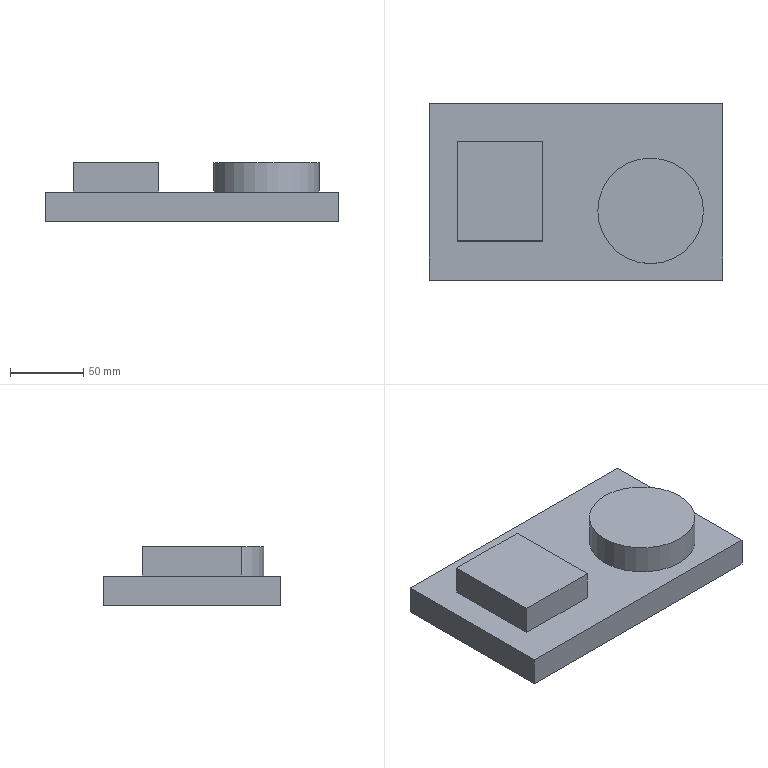CAM job | NX | mm | 3-axis | 1 set-up | 1 operations | part box 200 x 120 x 40
set-up 1
1. Face Milling | Mill MillChamfer D15R0 | FACE_MILLING | path 19258.324 mm | 31.533 min